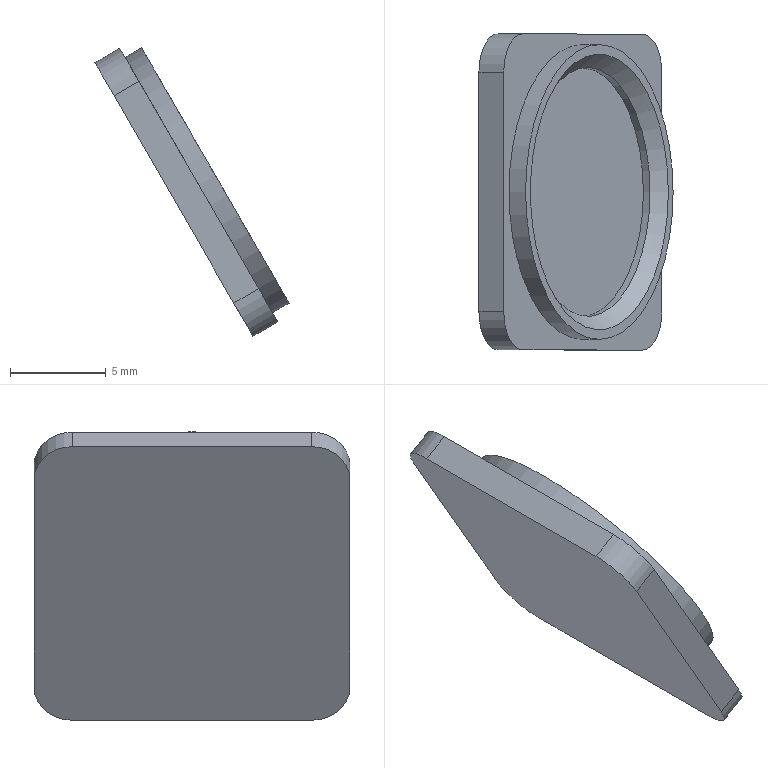Component | NX | ANALOG_FINGERPRINT_BUTTON | 1 solid | 15 faces | box 10.14 x 16.5 x 15.06 mm | volume 433 mm3 | plane 8 | cylinder 6 | cone 1 | commonest cylinder face diameters 4 x4 15.4 x1 13 x1
STEP:
#1=CARTESIAN_POINT('',(0.,0.,0.));
#2=DIRECTION('',(0.,0.,1.));
#3=DIRECTION('',(1.,0.,0.));
#4=AXIS2_PLACEMENT_3D('',#1,#2,#3);
#5=CARTESIAN_POINT('',(-17.256,7.851,157.651));
#6=VERTEX_POINT('',#5);
#7=CARTESIAN_POINT('',(-17.256,-4.649,157.651));
#8=VERTEX_POINT('',#7);
#9=CARTESIAN_POINT('',(-17.256,7.851,157.651));
#10=DIRECTION('',(0.,-1.,0.));
#11=VECTOR('',#10,1.);
#12=LINE('',#9,#11);
#13=CARTESIAN_POINT('',(-15.957,7.851,158.401));
#14=DIRECTION('',(0.5,0.,-0.866));
#15=DIRECTION('',(-0.866,0.,-0.5));
#16=AXIS2_PLACEMENT_3D('',#13,#14,#15);
#17=PLANE('',#16);
#18=CARTESIAN_POINT('',(1.5,0.));
#19=DIRECTION('',(0.,-1.));
#20=VECTOR('',#19,1.);
#21=LINE('',#18,#20);
#22=(GEOMETRIC_REPRESENTATION_CONTEXT(2)PARAMETRIC_REPRESENTATION_CONTEXT()REPRESENTATION_CONTEXT('',''));
#23=DEFINITIONAL_REPRESENTATION('',(#21),#22);
#24=PCURVE('',#17,#23);
#25=CARTESIAN_POINT('',(-16.256,-4.649,155.919));
#26=DIRECTION('',(0.866,0.,0.5));
#27=DIRECTION('',(0.5,0.,-0.866));
#28=AXIS2_PLACEMENT_3D('',#25,#26,#27);
#29=PLANE('',#28);
#30=CARTESIAN_POINT('',(-2.,12.5));
#31=DIRECTION('',(0.,-1.));
#32=VECTOR('',#31,1.);
#33=LINE('',#30,#32);
#34=(GEOMETRIC_REPRESENTATION_CONTEXT(2)PARAMETRIC_REPRESENTATION_CONTEXT()REPRESENTATION_CONTEXT('',''));
#35=DEFINITIONAL_REPRESENTATION('',(#33),#34);
#36=PCURVE('',#29,#35);
#37=SURFACE_CURVE('',#12,(#24,#36),.PCURVE_S1.);
#38=EDGE_CURVE('',#6,#8,#37,.T.);
#39=ORIENTED_EDGE('',*,*,#38,.T.);
#40=CARTESIAN_POINT('',(-15.957,-4.649,158.401));
#41=VERTEX_POINT('',#40);
#42=CARTESIAN_POINT('',(-15.957,-4.649,158.401));
#43=DIRECTION('',(-0.866,0.,-0.5));
#44=VECTOR('',#43,1.);
#45=LINE('',#42,#44);
#46=CARTESIAN_POINT('',(0.,-12.5));
#47=DIRECTION('',(1.,0.));
#48=VECTOR('',#47,1.);
#49=LINE('',#46,#48);
#50=(GEOMETRIC_REPRESENTATION_CONTEXT(2)PARAMETRIC_REPRESENTATION_CONTEXT()REPRESENTATION_CONTEXT('',''));
#51=DEFINITIONAL_REPRESENTATION('',(#49),#50);
#52=PCURVE('',#17,#51);
#53=CARTESIAN_POINT('',(-14.957,-4.649,156.669));
#54=DIRECTION('',(-0.866,0.,-0.5));
#55=DIRECTION('',(-0.5,0.,0.866));
#56=AXIS2_PLACEMENT_3D('',#53,#54,#55);
#57=CYLINDRICAL_SURFACE('',#56,2.);
#58=CARTESIAN_POINT('',(6.283,0.));
#59=DIRECTION('',(0.,1.));
#60=VECTOR('',#59,1.);
#61=LINE('',#58,#60);
#62=(GEOMETRIC_REPRESENTATION_CONTEXT(2)PARAMETRIC_REPRESENTATION_CONTEXT()REPRESENTATION_CONTEXT('',''));
#63=DEFINITIONAL_REPRESENTATION('',(#61),#62);
#64=PCURVE('',#57,#63);
#65=SURFACE_CURVE('',#45,(#52,#64),.PCURVE_S1.);
#66=EDGE_CURVE('',#41,#8,#65,.T.);
#67=ORIENTED_EDGE('',*,*,#66,.F.);
#68=CARTESIAN_POINT('',(-15.957,7.851,158.401));
#69=VERTEX_POINT('',#68);
#70=CARTESIAN_POINT('',(-15.957,7.851,158.401));
#71=DIRECTION('',(0.,-1.,0.));
#72=VECTOR('',#71,1.);
#73=LINE('',#70,#72);
#74=CARTESIAN_POINT('',(0.,0.));
#75=DIRECTION('',(0.,-1.));
#76=VECTOR('',#75,1.);
#77=LINE('',#74,#76);
#78=(GEOMETRIC_REPRESENTATION_CONTEXT(2)PARAMETRIC_REPRESENTATION_CONTEXT()REPRESENTATION_CONTEXT('',''));
#79=DEFINITIONAL_REPRESENTATION('',(#77),#78);
#80=PCURVE('',#17,#79);
#81=CARTESIAN_POINT('',(-14.957,-4.649,156.669));
#82=DIRECTION('',(0.866,0.,0.5));
#83=DIRECTION('',(0.5,0.,-0.866));
#84=AXIS2_PLACEMENT_3D('',#81,#82,#83);
#85=PLANE('',#84);
#86=CARTESIAN_POINT('',(-2.,12.5));
#87=DIRECTION('',(0.,-1.));
#88=VECTOR('',#87,1.);
#89=LINE('',#86,#88);
#90=(GEOMETRIC_REPRESENTATION_CONTEXT(2)PARAMETRIC_REPRESENTATION_CONTEXT()REPRESENTATION_CONTEXT('',''));
#91=DEFINITIONAL_REPRESENTATION('',(#89),#90);
#92=PCURVE('',#85,#91);
#93=SURFACE_CURVE('',#73,(#80,#92),.PCURVE_S1.);
#94=EDGE_CURVE('',#69,#41,#93,.T.);
#95=ORIENTED_EDGE('',*,*,#94,.F.);
#96=CARTESIAN_POINT('',(-15.957,7.851,158.401));
#97=DIRECTION('',(-0.866,0.,-0.5));
#98=VECTOR('',#97,1.);
#99=LINE('',#96,#98);
#100=CARTESIAN_POINT('',(0.,0.));
#101=DIRECTION('',(1.,0.));
#102=VECTOR('',#101,1.);
#103=LINE('',#100,#102);
#104=(GEOMETRIC_REPRESENTATION_CONTEXT(2)PARAMETRIC_REPRESENTATION_CONTEXT()REPRESENTATION_CONTEXT('',''));
#105=DEFINITIONAL_REPRESENTATION('',(#103),#104);
#106=PCURVE('',#17,#105);
#107=CARTESIAN_POINT('',(-14.957,7.851,156.669));
#108=DIRECTION('',(-0.866,0.,-0.5));
#109=DIRECTION('',(-0.5,0.,0.866));
#110=AXIS2_PLACEMENT_3D('',#107,#108,#109);
#111=CYLINDRICAL_SURFACE('',#110,2.);
#112=CARTESIAN_POINT('',(0.,0.));
#113=DIRECTION('',(0.,1.));
#114=VECTOR('',#113,1.);
#115=LINE('',#112,#114);
#116=(GEOMETRIC_REPRESENTATION_CONTEXT(2)PARAMETRIC_REPRESENTATION_CONTEXT()REPRESENTATION_CONTEXT('',''));
#117=DEFINITIONAL_REPRESENTATION('',(#115),#116);
#118=PCURVE('',#111,#117);
#119=SURFACE_CURVE('',#99,(#106,#118),.PCURVE_S1.);
#120=EDGE_CURVE('',#69,#6,#119,.T.);
#121=ORIENTED_EDGE('',*,*,#120,.T.);
#122=EDGE_LOOP('',(#39,#67,#95,#121));
#123=FACE_BOUND('',#122,.T.);
#124=ADVANCED_FACE('',(#123),#17,.F.);
#125=CARTESIAN_POINT('',(-16.256,-6.649,155.919));
#126=VERTEX_POINT('',#125);
#127=CARTESIAN_POINT('',(-16.256,-4.649,155.919));
#128=DIRECTION('',(0.866,0.,0.5));
#129=DIRECTION('',(0.5,0.,-0.866));
#130=AXIS2_PLACEMENT_3D('',#127,#128,#129);
#131=CIRCLE('',#130,2.);
#132=CARTESIAN_POINT('',(9.425,1.5));
#133=DIRECTION('',(-1.,-0.));
#134=VECTOR('',#133,1.);
#135=LINE('',#132,#134);
#136=(GEOMETRIC_REPRESENTATION_CONTEXT(2)PARAMETRIC_REPRESENTATION_CONTEXT()REPRESENTATION_CONTEXT('',''));
#137=DEFINITIONAL_REPRESENTATION('',(#135),#136);
#138=PCURVE('',#57,#137);
#139=CARTESIAN_POINT('',(0.,0.));
#140=DIRECTION('',(1.,0.));
#141=AXIS2_PLACEMENT_2D('',#139,#140);
#142=CIRCLE('',#141,2.);
#143=(GEOMETRIC_REPRESENTATION_CONTEXT(2)PARAMETRIC_REPRESENTATION_CONTEXT()REPRESENTATION_CONTEXT('',''));
#144=DEFINITIONAL_REPRESENTATION('',(#142),#143);
#145=PCURVE('',#29,#144);
#146=SURFACE_CURVE('',#131,(#138,#145),.PCURVE_S1.);
#147=EDGE_CURVE('',#8,#126,#146,.T.);
#148=ORIENTED_EDGE('',*,*,#147,.T.);
#149=CARTESIAN_POINT('',(-14.957,-6.649,156.669));
#150=VERTEX_POINT('',#149);
#151=CARTESIAN_POINT('',(-14.957,-6.649,156.669));
#152=DIRECTION('',(-0.866,0.,-0.5));
#153=VECTOR('',#152,1.);
#154=LINE('',#151,#153);
#155=CARTESIAN_POINT('',(4.712,0.));
#156=DIRECTION('',(0.,1.));
#157=VECTOR('',#156,1.);
#158=LINE('',#155,#157);
#159=(GEOMETRIC_REPRESENTATION_CONTEXT(2)PARAMETRIC_REPRESENTATION_CONTEXT()REPRESENTATION_CONTEXT('',''));
#160=DEFINITIONAL_REPRESENTATION('',(#158),#159);
#161=PCURVE('',#57,#160);
#162=CARTESIAN_POINT('',(-14.957,-6.649,156.669));
#163=DIRECTION('',(0.,1.,0.));
#164=DIRECTION('',(0.866,0.,0.5));
#165=AXIS2_PLACEMENT_3D('',#162,#163,#164);
#166=PLANE('',#165);
#167=CARTESIAN_POINT('',(0.,0.));
#168=DIRECTION('',(-1.,0.));
#169=VECTOR('',#168,1.);
#170=LINE('',#167,#169);
#171=(GEOMETRIC_REPRESENTATION_CONTEXT(2)PARAMETRIC_REPRESENTATION_CONTEXT()REPRESENTATION_CONTEXT('',''));
#172=DEFINITIONAL_REPRESENTATION('',(#170),#171);
#173=PCURVE('',#166,#172);
#174=SURFACE_CURVE('',#154,(#161,#173),.PCURVE_S1.);
#175=EDGE_CURVE('',#150,#126,#174,.T.);
#176=ORIENTED_EDGE('',*,*,#175,.F.);
#177=CARTESIAN_POINT('',(-14.957,-4.649,156.669));
#178=DIRECTION('',(0.866,0.,0.5));
#179=DIRECTION('',(0.5,0.,-0.866));
#180=AXIS2_PLACEMENT_3D('',#177,#178,#179);
#181=CIRCLE('',#180,2.);
#182=CARTESIAN_POINT('',(9.425,0.));
#183=DIRECTION('',(-1.,0.));
#184=VECTOR('',#183,1.);
#185=LINE('',#182,#184);
#186=(GEOMETRIC_REPRESENTATION_CONTEXT(2)PARAMETRIC_REPRESENTATION_CONTEXT()REPRESENTATION_CONTEXT('',''));
#187=DEFINITIONAL_REPRESENTATION('',(#185),#186);
#188=PCURVE('',#57,#187);
#189=CARTESIAN_POINT('',(0.,0.));
#190=DIRECTION('',(1.,0.));
#191=AXIS2_PLACEMENT_2D('',#189,#190);
#192=CIRCLE('',#191,2.);
#193=(GEOMETRIC_REPRESENTATION_CONTEXT(2)PARAMETRIC_REPRESENTATION_CONTEXT()REPRESENTATION_CONTEXT('',''));
#194=DEFINITIONAL_REPRESENTATION('',(#192),#193);
#195=PCURVE('',#85,#194);
#196=SURFACE_CURVE('',#181,(#188,#195),.PCURVE_S1.);
#197=EDGE_CURVE('',#41,#150,#196,.T.);
#198=ORIENTED_EDGE('',*,*,#197,.F.);
#199=ORIENTED_EDGE('',*,*,#66,.T.);
#200=EDGE_LOOP('',(#148,#176,#198,#199));
#201=FACE_BOUND('',#200,.T.);
#202=ADVANCED_FACE('',(#201),#57,.T.);
#203=CARTESIAN_POINT('',(-10.006,-6.649,145.094));
#204=VERTEX_POINT('',#203);
#205=CARTESIAN_POINT('',(-16.256,-6.649,155.919));
#206=DIRECTION('',(0.5,0.,-0.866));
#207=VECTOR('',#206,1.);
#208=LINE('',#205,#207);
#209=CARTESIAN_POINT('',(-1.5,0.));
#210=DIRECTION('',(0.,1.));
#211=VECTOR('',#210,1.);
#212=LINE('',#209,#211);
#213=(GEOMETRIC_REPRESENTATION_CONTEXT(2)PARAMETRIC_REPRESENTATION_CONTEXT()REPRESENTATION_CONTEXT('',''));
#214=DEFINITIONAL_REPRESENTATION('',(#212),#213);
#215=PCURVE('',#166,#214);
#216=CARTESIAN_POINT('',(0.,-2.));
#217=DIRECTION('',(1.,0.));
#218=VECTOR('',#217,1.);
#219=LINE('',#216,#218);
#220=(GEOMETRIC_REPRESENTATION_CONTEXT(2)PARAMETRIC_REPRESENTATION_CONTEXT()REPRESENTATION_CONTEXT('',''));
#221=DEFINITIONAL_REPRESENTATION('',(#219),#220);
#222=PCURVE('',#29,#221);
#223=SURFACE_CURVE('',#208,(#215,#222),.PCURVE_S1.);
#224=EDGE_CURVE('',#126,#204,#223,.T.);
#225=ORIENTED_EDGE('',*,*,#224,.T.);
#226=CARTESIAN_POINT('',(-8.707,-6.649,145.844));
#227=VERTEX_POINT('',#226);
#228=CARTESIAN_POINT('',(-8.707,-6.649,145.844));
#229=DIRECTION('',(-0.866,0.,-0.5));
#230=VECTOR('',#229,1.);
#231=LINE('',#228,#230);
#232=CARTESIAN_POINT('',(-0.,12.5));
#233=DIRECTION('',(-1.,0.));
#234=VECTOR('',#233,1.);
#235=LINE('',#232,#234);
#236=(GEOMETRIC_REPRESENTATION_CONTEXT(2)PARAMETRIC_REPRESENTATION_CONTEXT()REPRESENTATION_CONTEXT('',''));
#237=DEFINITIONAL_REPRESENTATION('',(#235),#236);
#238=PCURVE('',#166,#237);
#239=CARTESIAN_POINT('',(-8.707,-4.649,145.844));
#240=DIRECTION('',(-0.866,0.,-0.5));
#241=DIRECTION('',(-0.5,0.,0.866));
#242=AXIS2_PLACEMENT_3D('',#239,#240,#241);
#243=CYLINDRICAL_SURFACE('',#242,2.);
#244=CARTESIAN_POINT('',(4.712,0.));
#245=DIRECTION('',(0.,1.));
#246=VECTOR('',#245,1.);
#247=LINE('',#244,#246);
#248=(GEOMETRIC_REPRESENTATION_CONTEXT(2)PARAMETRIC_REPRESENTATION_CONTEXT()REPRESENTATION_CONTEXT('',''));
#249=DEFINITIONAL_REPRESENTATION('',(#247),#248);
#250=PCURVE('',#243,#249);
#251=SURFACE_CURVE('',#231,(#238,#250),.PCURVE_S1.);
#252=EDGE_CURVE('',#227,#204,#251,.T.);
#253=ORIENTED_EDGE('',*,*,#252,.F.);
#254=CARTESIAN_POINT('',(-14.957,-6.649,156.669));
#255=DIRECTION('',(0.5,0.,-0.866));
#256=VECTOR('',#255,1.);
#257=LINE('',#254,#256);
#258=CARTESIAN_POINT('',(0.,0.));
#259=DIRECTION('',(0.,1.));
#260=VECTOR('',#259,1.);
#261=LINE('',#258,#260);
#262=(GEOMETRIC_REPRESENTATION_CONTEXT(2)PARAMETRIC_REPRESENTATION_CONTEXT()REPRESENTATION_CONTEXT('',''));
#263=DEFINITIONAL_REPRESENTATION('',(#261),#262);
#264=PCURVE('',#166,#263);
#265=CARTESIAN_POINT('',(0.,-2.));
#266=DIRECTION('',(1.,0.));
#267=VECTOR('',#266,1.);
#268=LINE('',#265,#267);
#269=(GEOMETRIC_REPRESENTATION_CONTEXT(2)PARAMETRIC_REPRESENTATION_CONTEXT()REPRESENTATION_CONTEXT('',''));
#270=DEFINITIONAL_REPRESENTATION('',(#268),#269);
#271=PCURVE('',#85,#270);
#272=SURFACE_CURVE('',#257,(#264,#271),.PCURVE_S1.);
#273=EDGE_CURVE('',#150,#227,#272,.T.);
#274=ORIENTED_EDGE('',*,*,#273,.F.);
#275=ORIENTED_EDGE('',*,*,#175,.T.);
#276=EDGE_LOOP('',(#225,#253,#274,#275));
#277=FACE_BOUND('',#276,.T.);
#278=ADVANCED_FACE('',(#277),#166,.F.);
#279=CARTESIAN_POINT('',(-9.006,-4.649,143.362));
#280=VERTEX_POINT('',#279);
#281=CARTESIAN_POINT('',(-10.006,-4.649,145.094));
#282=DIRECTION('',(0.866,0.,0.5));
#283=DIRECTION('',(0.5,0.,-0.866));
#284=AXIS2_PLACEMENT_3D('',#281,#282,#283);
#285=CIRCLE('',#284,2.);
#286=CARTESIAN_POINT('',(9.425,1.5));
#287=DIRECTION('',(-1.,0.));
#288=VECTOR('',#287,1.);
#289=LINE('',#286,#288);
#290=(GEOMETRIC_REPRESENTATION_CONTEXT(2)PARAMETRIC_REPRESENTATION_CONTEXT()REPRESENTATION_CONTEXT('',''));
#291=DEFINITIONAL_REPRESENTATION('',(#289),#290);
#292=PCURVE('',#243,#291);
#293=CARTESIAN_POINT('',(12.5,0.));
#294=DIRECTION('',(1.,0.));
#295=AXIS2_PLACEMENT_2D('',#293,#294);
#296=CIRCLE('',#295,2.);
#297=(GEOMETRIC_REPRESENTATION_CONTEXT(2)PARAMETRIC_REPRESENTATION_CONTEXT()REPRESENTATION_CONTEXT('',''));
#298=DEFINITIONAL_REPRESENTATION('',(#296),#297);
#299=PCURVE('',#29,#298);
#300=SURFACE_CURVE('',#285,(#292,#299),.PCURVE_S1.);
#301=EDGE_CURVE('',#204,#280,#300,.T.);
#302=ORIENTED_EDGE('',*,*,#301,.T.);
#303=CARTESIAN_POINT('',(-7.707,-4.649,144.112));
#304=VERTEX_POINT('',#303);
#305=CARTESIAN_POINT('',(-7.707,-4.649,144.112));
#306=DIRECTION('',(-0.866,0.,-0.5));
#307=VECTOR('',#306,1.);
#308=LINE('',#305,#307);
#309=CARTESIAN_POINT('',(3.142,0.));
#310=DIRECTION('',(0.,1.));
#311=VECTOR('',#310,1.);
#312=LINE('',#309,#311);
#313=(GEOMETRIC_REPRESENTATION_CONTEXT(2)PARAMETRIC_REPRESENTATION_CONTEXT()REPRESENTATION_CONTEXT('',''));
#314=DEFINITIONAL_REPRESENTATION('',(#312),#313);
#315=PCURVE('',#243,#314);
#316=CARTESIAN_POINT('',(-7.707,-4.649,144.112));
#317=DIRECTION('',(-0.5,0.,0.866));
#318=DIRECTION('',(0.866,0.,0.5));
#319=AXIS2_PLACEMENT_3D('',#316,#317,#318);
#320=PLANE('',#319);
#321=CARTESIAN_POINT('',(0.,0.));
#322=DIRECTION('',(-1.,0.));
#323=VECTOR('',#322,1.);
#324=LINE('',#321,#323);
#325=(GEOMETRIC_REPRESENTATION_CONTEXT(2)PARAMETRIC_REPRESENTATION_CONTEXT()REPRESENTATION_CONTEXT('',''));
#326=DEFINITIONAL_REPRESENTATION('',(#324),#325);
#327=PCURVE('',#320,#326);
#328=SURFACE_CURVE('',#308,(#315,#327),.PCURVE_S1.);
#329=EDGE_CURVE('',#304,#280,#328,.T.);
#330=ORIENTED_EDGE('',*,*,#329,.F.);
#331=CARTESIAN_POINT('',(-8.707,-4.649,145.844));
#332=DIRECTION('',(0.866,0.,0.5));
#333=DIRECTION('',(0.5,0.,-0.866));
#334=AXIS2_PLACEMENT_3D('',#331,#332,#333);
#335=CIRCLE('',#334,2.);
#336=CARTESIAN_POINT('',(9.425,0.));
#337=DIRECTION('',(-1.,-0.));
#338=VECTOR('',#337,1.);
#339=LINE('',#336,#338);
#340=(GEOMETRIC_REPRESENTATION_CONTEXT(2)PARAMETRIC_REPRESENTATION_CONTEXT()REPRESENTATION_CONTEXT('',''));
#341=DEFINITIONAL_REPRESENTATION('',(#339),#340);
#342=PCURVE('',#243,#341);
#343=CARTESIAN_POINT('',(12.5,0.));
#344=DIRECTION('',(1.,0.));
#345=AXIS2_PLACEMENT_2D('',#343,#344);
#346=CIRCLE('',#345,2.);
#347=(GEOMETRIC_REPRESENTATION_CONTEXT(2)PARAMETRIC_REPRESENTATION_CONTEXT()REPRESENTATION_CONTEXT('',''));
#348=DEFINITIONAL_REPRESENTATION('',(#346),#347);
#349=PCURVE('',#85,#348);
#350=SURFACE_CURVE('',#335,(#342,#349),.PCURVE_S1.);
#351=EDGE_CURVE('',#227,#304,#350,.T.);
#352=ORIENTED_EDGE('',*,*,#351,.F.);
#353=ORIENTED_EDGE('',*,*,#252,.T.);
#354=EDGE_LOOP('',(#302,#330,#352,#353));
#355=FACE_BOUND('',#354,.T.);
#356=ADVANCED_FACE('',(#355),#243,.T.);
#357=CARTESIAN_POINT('',(-9.006,7.851,143.362));
#358=VERTEX_POINT('',#357);
#359=CARTESIAN_POINT('',(-9.006,-4.649,143.362));
#360=DIRECTION('',(0.,1.,0.));
#361=VECTOR('',#360,1.);
#362=LINE('',#359,#361);
#363=CARTESIAN_POINT('',(-1.5,0.));
#364=DIRECTION('',(0.,1.));
#365=VECTOR('',#364,1.);
#366=LINE('',#363,#365);
#367=(GEOMETRIC_REPRESENTATION_CONTEXT(2)PARAMETRIC_REPRESENTATION_CONTEXT()REPRESENTATION_CONTEXT('',''));
#368=DEFINITIONAL_REPRESENTATION('',(#366),#367);
#369=PCURVE('',#320,#368);
#370=CARTESIAN_POINT('',(14.5,0.));
#371=DIRECTION('',(0.,1.));
#372=VECTOR('',#371,1.);
#373=LINE('',#370,#372);
#374=(GEOMETRIC_REPRESENTATION_CONTEXT(2)PARAMETRIC_REPRESENTATION_CONTEXT()REPRESENTATION_CONTEXT('',''));
#375=DEFINITIONAL_REPRESENTATION('',(#373),#374);
#376=PCURVE('',#29,#375);
#377=SURFACE_CURVE('',#362,(#369,#376),.PCURVE_S1.);
#378=EDGE_CURVE('',#280,#358,#377,.T.);
#379=ORIENTED_EDGE('',*,*,#378,.T.);
#380=CARTESIAN_POINT('',(-7.707,7.851,144.112));
#381=VERTEX_POINT('',#380);
#382=CARTESIAN_POINT('',(-7.707,7.851,144.112));
#383=DIRECTION('',(-0.866,0.,-0.5));
#384=VECTOR('',#383,1.);
#385=LINE('',#382,#384);
#386=CARTESIAN_POINT('',(0.,12.5));
#387=DIRECTION('',(-1.,0.));
#388=VECTOR('',#387,1.);
#389=LINE('',#386,#388);
#390=(GEOMETRIC_REPRESENTATION_CONTEXT(2)PARAMETRIC_REPRESENTATION_CONTEXT()REPRESENTATION_CONTEXT('',''));
#391=DEFINITIONAL_REPRESENTATION('',(#389),#390);
#392=PCURVE('',#320,#391);
#393=CARTESIAN_POINT('',(-8.707,7.851,145.844));
#394=DIRECTION('',(-0.866,0.,-0.5));
#395=DIRECTION('',(-0.5,0.,0.866));
#396=AXIS2_PLACEMENT_3D('',#393,#394,#395);
#397=CYLINDRICAL_SURFACE('',#396,2.);
#398=CARTESIAN_POINT('',(3.142,0.));
#399=DIRECTION('',(0.,1.));
#400=VECTOR('',#399,1.);
#401=LINE('',#398,#400);
#402=(GEOMETRIC_REPRESENTATION_CONTEXT(2)PARAMETRIC_REPRESENTATION_CONTEXT()REPRESENTATION_CONTEXT('',''));
#403=DEFINITIONAL_REPRESENTATION('',(#401),#402);
#404=PCURVE('',#397,#403);
#405=SURFACE_CURVE('',#385,(#392,#404),.PCURVE_S1.);
#406=EDGE_CURVE('',#381,#358,#405,.T.);
#407=ORIENTED_EDGE('',*,*,#406,.F.);
#408=CARTESIAN_POINT('',(-7.707,-4.649,144.112));
#409=DIRECTION('',(0.,1.,0.));
#410=VECTOR('',#409,1.);
#411=LINE('',#408,#410);
#412=CARTESIAN_POINT('',(0.,0.));
#413=DIRECTION('',(0.,1.));
#414=VECTOR('',#413,1.);
#415=LINE('',#412,#414);
#416=(GEOMETRIC_REPRESENTATION_CONTEXT(2)PARAMETRIC_REPRESENTATION_CONTEXT()REPRESENTATION_CONTEXT('',''));
#417=DEFINITIONAL_REPRESENTATION('',(#415),#416);
#418=PCURVE('',#320,#417);
#419=CARTESIAN_POINT('',(14.5,0.));
#420=DIRECTION('',(0.,1.));
#421=VECTOR('',#420,1.);
#422=LINE('',#419,#421);
#423=(GEOMETRIC_REPRESENTATION_CONTEXT(2)PARAMETRIC_REPRESENTATION_CONTEXT()REPRESENTATION_CONTEXT('',''));
#424=DEFINITIONAL_REPRESENTATION('',(#422),#423);
#425=PCURVE('',#85,#424);
#426=SURFACE_CURVE('',#411,(#418,#425),.PCURVE_S1.);
#427=EDGE_CURVE('',#304,#381,#426,.T.);
#428=ORIENTED_EDGE('',*,*,#427,.F.);
#429=ORIENTED_EDGE('',*,*,#329,.T.);
#430=EDGE_LOOP('',(#379,#407,#428,#429));
#431=FACE_BOUND('',#430,.T.);
#432=ADVANCED_FACE('',(#431),#320,.F.);
#433=CARTESIAN_POINT('',(-10.006,9.851,145.094));
#434=VERTEX_POINT('',#433);
#435=CARTESIAN_POINT('',(-10.006,7.851,145.094));
#436=DIRECTION('',(0.866,0.,0.5));
#437=DIRECTION('',(0.5,0.,-0.866));
#438=AXIS2_PLACEMENT_3D('',#435,#436,#437);
#439=CIRCLE('',#438,2.);
#440=CARTESIAN_POINT('',(3.142,1.5));
#441=DIRECTION('',(-1.,0.));
#442=VECTOR('',#441,1.);
#443=LINE('',#440,#442);
#444=(GEOMETRIC_REPRESENTATION_CONTEXT(2)PARAMETRIC_REPRESENTATION_CONTEXT()REPRESENTATION_CONTEXT('',''));
#445=DEFINITIONAL_REPRESENTATION('',(#443),#444);
#446=PCURVE('',#397,#445);
#447=CARTESIAN_POINT('',(12.5,12.5));
#448=DIRECTION('',(1.,0.));
#449=AXIS2_PLACEMENT_2D('',#447,#448);
#450=CIRCLE('',#449,2.);
#451=(GEOMETRIC_REPRESENTATION_CONTEXT(2)PARAMETRIC_REPRESENTATION_CONTEXT()REPRESENTATION_CONTEXT('',''));
#452=DEFINITIONAL_REPRESENTATION('',(#450),#451);
#453=PCURVE('',#29,#452);
#454=SURFACE_CURVE('',#439,(#446,#453),.PCURVE_S1.);
#455=EDGE_CURVE('',#358,#434,#454,.T.);
#456=ORIENTED_EDGE('',*,*,#455,.T.);
#457=CARTESIAN_POINT('',(-8.707,9.851,145.844));
#458=VERTEX_POINT('',#457);
#459=CARTESIAN_POINT('',(-8.707,9.851,145.844));
#460=DIRECTION('',(-0.866,0.,-0.5));
#461=VECTOR('',#460,1.);
#462=LINE('',#459,#461);
#463=CARTESIAN_POINT('',(1.571,0.));
#464=DIRECTION('',(-0.,1.));
#465=VECTOR('',#464,1.);
#466=LINE('',#463,#465);
#467=(GEOMETRIC_REPRESENTATION_CONTEXT(2)PARAMETRIC_REPRESENTATION_CONTEXT()REPRESENTATION_CONTEXT('',''));
#468=DEFINITIONAL_REPRESENTATION('',(#466),#467);
#469=PCURVE('',#397,#468);
#470=CARTESIAN_POINT('',(-8.707,9.851,145.844));
#471=DIRECTION('',(0.,-1.,0.));
#472=DIRECTION('',(-0.866,0.,-0.5));
#473=AXIS2_PLACEMENT_3D('',#470,#471,#472);
#474=PLANE('',#473);
#475=CARTESIAN_POINT('',(0.,0.));
#476=DIRECTION('',(1.,0.));
#477=VECTOR('',#476,1.);
#478=LINE('',#475,#477);
#479=(GEOMETRIC_REPRESENTATION_CONTEXT(2)PARAMETRIC_REPRESENTATION_CONTEXT()REPRESENTATION_CONTEXT('',''));
#480=DEFINITIONAL_REPRESENTATION('',(#478),#479);
#481=PCURVE('',#474,#480);
#482=SURFACE_CURVE('',#462,(#469,#481),.PCURVE_S1.);
#483=EDGE_CURVE('',#458,#434,#482,.T.);
#484=ORIENTED_EDGE('',*,*,#483,.F.);
#485=CARTESIAN_POINT('',(-8.707,7.851,145.844));
#486=DIRECTION('',(0.866,0.,0.5));
#487=DIRECTION('',(0.5,0.,-0.866));
#488=AXIS2_PLACEMENT_3D('',#485,#486,#487);
#489=CIRCLE('',#488,2.);
#490=CARTESIAN_POINT('',(3.142,-0.));
#491=DIRECTION('',(-1.,0.));
#492=VECTOR('',#491,1.);
#493=LINE('',#490,#492);
#494=(GEOMETRIC_REPRESENTATION_CONTEXT(2)PARAMETRIC_REPRESENTATION_CONTEXT()REPRESENTATION_CONTEXT('',''));
#495=DEFINITIONAL_REPRESENTATION('',(#493),#494);
#496=PCURVE('',#397,#495);
#497=CARTESIAN_POINT('',(12.5,12.5));
#498=DIRECTION('',(1.,0.));
#499=AXIS2_PLACEMENT_2D('',#497,#498);
#500=CIRCLE('',#499,2.);
#501=(GEOMETRIC_REPRESENTATION_CONTEXT(2)PARAMETRIC_REPRESENTATION_CONTEXT()REPRESENTATION_CONTEXT('',''));
#502=DEFINITIONAL_REPRESENTATION('',(#500),#501);
#503=PCURVE('',#85,#502);
#504=SURFACE_CURVE('',#489,(#496,#503),.PCURVE_S1.);
#505=EDGE_CURVE('',#381,#458,#504,.T.);
#506=ORIENTED_EDGE('',*,*,#505,.F.);
#507=ORIENTED_EDGE('',*,*,#406,.T.);
#508=EDGE_LOOP('',(#456,#484,#506,#507));
#509=FACE_BOUND('',#508,.T.);
#510=ADVANCED_FACE('',(#509),#397,.T.);
#511=CARTESIAN_POINT('',(-16.256,9.851,155.919));
#512=VERTEX_POINT('',#511);
#513=CARTESIAN_POINT('',(-10.006,9.851,145.094));
#514=DIRECTION('',(-0.5,0.,0.866));
#515=VECTOR('',#514,1.);
#516=LINE('',#513,#515);
#517=CARTESIAN_POINT('',(1.5,0.));
#518=DIRECTION('',(0.,-1.));
#519=VECTOR('',#518,1.);
#520=LINE('',#517,#519);
#521=(GEOMETRIC_REPRESENTATION_CONTEXT(2)PARAMETRIC_REPRESENTATION_CONTEXT()REPRESENTATION_CONTEXT('',''));
#522=DEFINITIONAL_REPRESENTATION('',(#520),#521);
#523=PCURVE('',#474,#522);
#524=CARTESIAN_POINT('',(12.5,14.5));
#525=DIRECTION('',(-1.,0.));
#526=VECTOR('',#525,1.);
#527=LINE('',#524,#526);
#528=(GEOMETRIC_REPRESENTATION_CONTEXT(2)PARAMETRIC_REPRESENTATION_CONTEXT()REPRESENTATION_CONTEXT('',''));
#529=DEFINITIONAL_REPRESENTATION('',(#527),#528);
#530=PCURVE('',#29,#529);
#531=SURFACE_CURVE('',#516,(#523,#530),.PCURVE_S1.);
#532=EDGE_CURVE('',#434,#512,#531,.T.);
#533=ORIENTED_EDGE('',*,*,#532,.T.);
#534=CARTESIAN_POINT('',(-14.957,9.851,156.669));
#535=VERTEX_POINT('',#534);
#536=CARTESIAN_POINT('',(-14.957,9.851,156.669));
#537=DIRECTION('',(-0.866,0.,-0.5));
#538=VECTOR('',#537,1.);
#539=LINE('',#536,#538);
#540=CARTESIAN_POINT('',(-0.,-12.5));
#541=DIRECTION('',(1.,0.));
#542=VECTOR('',#541,1.);
#543=LINE('',#540,#542);
#544=(GEOMETRIC_REPRESENTATION_CONTEXT(2)PARAMETRIC_REPRESENTATION_CONTEXT()REPRESENTATION_CONTEXT('',''));
#545=DEFINITIONAL_REPRESENTATION('',(#543),#544);
#546=PCURVE('',#474,#545);
#547=CARTESIAN_POINT('',(1.571,0.));
#548=DIRECTION('',(0.,1.));
#549=VECTOR('',#548,1.);
#550=LINE('',#547,#549);
#551=(GEOMETRIC_REPRESENTATION_CONTEXT(2)PARAMETRIC_REPRESENTATION_CONTEXT()REPRESENTATION_CONTEXT('',''));
#552=DEFINITIONAL_REPRESENTATION('',(#550),#551);
#553=PCURVE('',#111,#552);
#554=SURFACE_CURVE('',#539,(#546,#553),.PCURVE_S1.);
#555=EDGE_CURVE('',#535,#512,#554,.T.);
#556=ORIENTED_EDGE('',*,*,#555,.F.);
#557=CARTESIAN_POINT('',(-8.707,9.851,145.844));
#558=DIRECTION('',(-0.5,0.,0.866));
#559=VECTOR('',#558,1.);
#560=LINE('',#557,#559);
#561=CARTESIAN_POINT('',(0.,0.));
#562=DIRECTION('',(0.,-1.));
#563=VECTOR('',#562,1.);
#564=LINE('',#561,#563);
#565=(GEOMETRIC_REPRESENTATION_CONTEXT(2)PARAMETRIC_REPRESENTATION_CONTEXT()REPRESENTATION_CONTEXT('',''));
#566=DEFINITIONAL_REPRESENTATION('',(#564),#565);
#567=PCURVE('',#474,#566);
#568=CARTESIAN_POINT('',(12.5,14.5));
#569=DIRECTION('',(-1.,0.));
#570=VECTOR('',#569,1.);
#571=LINE('',#568,#570);
#572=(GEOMETRIC_REPRESENTATION_CONTEXT(2)PARAMETRIC_REPRESENTATION_CONTEXT()REPRESENTATION_CONTEXT('',''));
#573=DEFINITIONAL_REPRESENTATION('',(#571),#572);
#574=PCURVE('',#85,#573);
#575=SURFACE_CURVE('',#560,(#567,#574),.PCURVE_S1.);
#576=EDGE_CURVE('',#458,#535,#575,.T.);
#577=ORIENTED_EDGE('',*,*,#576,.F.);
#578=ORIENTED_EDGE('',*,*,#483,.T.);
#579=EDGE_LOOP('',(#533,#556,#577,#578));
#580=FACE_BOUND('',#579,.T.);
#581=ADVANCED_FACE('',(#580),#474,.F.);
#582=CARTESIAN_POINT('',(-16.256,7.851,155.919));
#583=DIRECTION('',(0.866,0.,0.5));
#584=DIRECTION('',(0.5,0.,-0.866));
#585=AXIS2_PLACEMENT_3D('',#582,#583,#584);
#586=CIRCLE('',#585,2.);
#587=CARTESIAN_POINT('',(3.142,1.5));
#588=DIRECTION('',(-1.,0.));
#589=VECTOR('',#588,1.);
#590=LINE('',#587,#589);
#591=(GEOMETRIC_REPRESENTATION_CONTEXT(2)PARAMETRIC_REPRESENTATION_CONTEXT()REPRESENTATION_CONTEXT('',''));
#592=DEFINITIONAL_REPRESENTATION('',(#590),#591);
#593=PCURVE('',#111,#592);
#594=CARTESIAN_POINT('',(0.,12.5));
#595=DIRECTION('',(1.,0.));
#596=AXIS2_PLACEMENT_2D('',#594,#595);
#597=CIRCLE('',#596,2.);
#598=(GEOMETRIC_REPRESENTATION_CONTEXT(2)PARAMETRIC_REPRESENTATION_CONTEXT()REPRESENTATION_CONTEXT('',''));
#599=DEFINITIONAL_REPRESENTATION('',(#597),#598);
#600=PCURVE('',#29,#599);
#601=SURFACE_CURVE('',#586,(#593,#600),.PCURVE_S1.);
#602=EDGE_CURVE('',#512,#6,#601,.T.);
#603=ORIENTED_EDGE('',*,*,#602,.T.);
#604=ORIENTED_EDGE('',*,*,#120,.F.);
#605=CARTESIAN_POINT('',(-14.957,7.851,156.669));
#606=DIRECTION('',(0.866,0.,0.5));
#607=DIRECTION('',(0.5,0.,-0.866));
#608=AXIS2_PLACEMENT_3D('',#605,#606,#607);
#609=CIRCLE('',#608,2.);
#610=CARTESIAN_POINT('',(3.142,0.));
#611=DIRECTION('',(-1.,0.));
#612=VECTOR('',#611,1.);
#613=LINE('',#610,#612);
#614=(GEOMETRIC_REPRESENTATION_CONTEXT(2)PARAMETRIC_REPRESENTATION_CONTEXT()REPRESENTATION_CONTEXT('',''));
#615=DEFINITIONAL_REPRESENTATION('',(#613),#614);
#616=PCURVE('',#111,#615);
#617=CARTESIAN_POINT('',(0.,12.5));
#618=DIRECTION('',(1.,0.));
#619=AXIS2_PLACEMENT_2D('',#617,#618);
#620=CIRCLE('',#619,2.);
#621=(GEOMETRIC_REPRESENTATION_CONTEXT(2)PARAMETRIC_REPRESENTATION_CONTEXT()REPRESENTATION_CONTEXT('',''));
#622=DEFINITIONAL_REPRESENTATION('',(#620),#621);
#623=PCURVE('',#85,#622);
#624=SURFACE_CURVE('',#609,(#616,#623),.PCURVE_S1.);
#625=EDGE_CURVE('',#535,#69,#624,.T.);
#626=ORIENTED_EDGE('',*,*,#625,.F.);
#627=ORIENTED_EDGE('',*,*,#555,.T.);
#628=EDGE_LOOP('',(#603,#604,#626,#627));
#629=FACE_BOUND('',#628,.T.);
#630=ADVANCED_FACE('',(#629),#111,.T.);
#631=CARTESIAN_POINT('',(-7.982,1.601,144.588));
#632=VERTEX_POINT('',#631);
#633=CARTESIAN_POINT('',(-11.832,1.601,151.257));
#634=DIRECTION('',(0.866,0.,0.5));
#635=DIRECTION('',(0.5,0.,-0.866));
#636=AXIS2_PLACEMENT_3D('',#633,#634,#635);
#637=CIRCLE('',#636,7.7);
#638=CARTESIAN_POINT('',(6.25,6.25));
#639=DIRECTION('',(1.,0.));
#640=AXIS2_PLACEMENT_2D('',#638,#639);
#641=CIRCLE('',#640,7.7);
#642=(GEOMETRIC_REPRESENTATION_CONTEXT(2)PARAMETRIC_REPRESENTATION_CONTEXT()REPRESENTATION_CONTEXT('',''));
#643=DEFINITIONAL_REPRESENTATION('',(#641),#642);
#644=PCURVE('',#85,#643);
#645=CARTESIAN_POINT('',(-13.131,1.601,150.507));
#646=DIRECTION('',(0.866,0.,0.5));
#647=DIRECTION('',(0.5,0.,-0.866));
#648=AXIS2_PLACEMENT_3D('',#645,#646,#647);
#649=CYLINDRICAL_SURFACE('',#648,7.7);
#650=CARTESIAN_POINT('',(0.,1.5));
#651=DIRECTION('',(1.,0.));
#652=VECTOR('',#651,1.);
#653=LINE('',#650,#652);
#654=(GEOMETRIC_REPRESENTATION_CONTEXT(2)PARAMETRIC_REPRESENTATION_CONTEXT()REPRESENTATION_CONTEXT('',''));
#655=DEFINITIONAL_REPRESENTATION('',(#653),#654);
#656=PCURVE('',#649,#655);
#657=SURFACE_CURVE('',#637,(#644,#656),.PCURVE_S1.);
#658=EDGE_CURVE('',#632,#632,#657,.T.);
#659=ORIENTED_EDGE('',*,*,#658,.F.);
#660=EDGE_LOOP('',(#659));
#661=FACE_BOUND('',#660,.T.);
#662=ORIENTED_EDGE('',*,*,#94,.T.);
#663=ORIENTED_EDGE('',*,*,#197,.T.);
#664=ORIENTED_EDGE('',*,*,#273,.T.);
#665=ORIENTED_EDGE('',*,*,#351,.T.);
#666=ORIENTED_EDGE('',*,*,#427,.T.);
#667=ORIENTED_EDGE('',*,*,#505,.T.);
#668=ORIENTED_EDGE('',*,*,#576,.T.);
#669=ORIENTED_EDGE('',*,*,#625,.T.);
#670=EDGE_LOOP('',(#662,#663,#664,#665,#666,#667,#668,#669));
#671=FACE_BOUND('',#670,.T.);
#672=ADVANCED_FACE('',(#661,#671),#85,.T.);
#673=ORIENTED_EDGE('',*,*,#38,.F.);
#674=ORIENTED_EDGE('',*,*,#602,.F.);
#675=ORIENTED_EDGE('',*,*,#532,.F.);
#676=ORIENTED_EDGE('',*,*,#455,.F.);
#677=ORIENTED_EDGE('',*,*,#378,.F.);
#678=ORIENTED_EDGE('',*,*,#301,.F.);
#679=ORIENTED_EDGE('',*,*,#224,.F.);
#680=ORIENTED_EDGE('',*,*,#147,.F.);
#681=EDGE_LOOP('',(#673,#674,#675,#676,#677,#678,#679,#680));
#682=FACE_BOUND('',#681,.T.);
#683=ADVANCED_FACE('',(#682),#29,.F.);
#684=CARTESIAN_POINT('',(-7.366,1.601,145.521));
#685=VERTEX_POINT('',#684);
#686=CARTESIAN_POINT('',(-10.966,1.601,151.757));
#687=DIRECTION('',(-0.866,0.,-0.5));
#688=DIRECTION('',(0.5,0.,-0.866));
#689=AXIS2_PLACEMENT_3D('',#686,#687,#688);
#690=CIRCLE('',#689,7.2);
#691=CARTESIAN_POINT('',(-10.966,1.601,151.757));
#692=DIRECTION('',(0.866,0.,0.5));
#693=DIRECTION('',(0.5,0.,-0.866));
#694=AXIS2_PLACEMENT_3D('',#691,#692,#693);
#695=PLANE('',#694);
#696=CARTESIAN_POINT('',(7.2,0.));
#697=CARTESIAN_POINT('',(7.2,-12.471));
#698=CARTESIAN_POINT('',(-3.6,-6.235));
#699=CARTESIAN_POINT('',(-14.4,-0.));
#700=CARTESIAN_POINT('',(-3.6,6.235));
#701=CARTESIAN_POINT('',(7.2,12.471));
#702=CARTESIAN_POINT('',(7.2,0.));
#703=(BOUNDED_CURVE()B_SPLINE_CURVE(2,(#696,#697,#698,#699,#700,#701,#702),.UNSPECIFIED.,.T.,.F.)B_SPLINE_CURVE_WITH_KNOTS((1,2,2,2,2,1),(-2.094,0.,2.094,4.189,6.283,8.378),.UNSPECIFIED.)CURVE()GEOMETRIC_REPRESENTATION_ITEM()RATIONAL_B_SPLINE_CURVE((1.,0.5,1.,0.5,1.,0.5,1.))REPRESENTATION_ITEM(''));
#704=(GEOMETRIC_REPRESENTATION_CONTEXT(2)PARAMETRIC_REPRESENTATION_CONTEXT()REPRESENTATION_CONTEXT('',''));
#705=DEFINITIONAL_REPRESENTATION('',(#703),#704);
#706=PCURVE('',#695,#705);
#707=CARTESIAN_POINT('',(-10.966,1.601,151.757));
#708=DIRECTION('',(0.866,0.,0.5));
#709=DIRECTION('',(0.5,0.,-0.866));
#710=AXIS2_PLACEMENT_3D('',#707,#708,#709);
#711=CONICAL_SURFACE('',#710,7.2,0.7854);
#712=CARTESIAN_POINT('',(6.283,0.));
#713=DIRECTION('',(-1.,0.));
#714=VECTOR('',#713,1.);
#715=LINE('',#712,#714);
#716=(GEOMETRIC_REPRESENTATION_CONTEXT(2)PARAMETRIC_REPRESENTATION_CONTEXT()REPRESENTATION_CONTEXT('',''));
#717=DEFINITIONAL_REPRESENTATION('',(#715),#716);
#718=PCURVE('',#711,#717);
#719=SURFACE_CURVE('',#690,(#706,#718),.PCURVE_S1.);
#720=EDGE_CURVE('',#685,#685,#719,.T.);
#721=ORIENTED_EDGE('',*,*,#720,.T.);
#722=EDGE_LOOP('',(#721));
#723=FACE_BOUND('',#722,.T.);
#724=CARTESIAN_POINT('',(-7.116,1.601,145.088));
#725=VERTEX_POINT('',#724);
#726=CARTESIAN_POINT('',(-10.966,1.601,151.757));
#727=DIRECTION('',(-0.866,0.,-0.5));
#728=DIRECTION('',(0.5,0.,-0.866));
#729=AXIS2_PLACEMENT_3D('',#726,#727,#728);
#730=CIRCLE('',#729,7.7);
#731=CARTESIAN_POINT('',(7.7,0.));
#732=CARTESIAN_POINT('',(7.7,-13.337));
#733=CARTESIAN_POINT('',(-3.85,-6.668));
#734=CARTESIAN_POINT('',(-15.4,-0.));
#735=CARTESIAN_POINT('',(-3.85,6.668));
#736=CARTESIAN_POINT('',(7.7,13.337));
#737=CARTESIAN_POINT('',(7.7,0.));
#738=(BOUNDED_CURVE()B_SPLINE_CURVE(2,(#731,#732,#733,#734,#735,#736,#737),.UNSPECIFIED.,.T.,.F.)B_SPLINE_CURVE_WITH_KNOTS((1,2,2,2,2,1),(-2.094,0.,2.094,4.189,6.283,8.378),.UNSPECIFIED.)CURVE()GEOMETRIC_REPRESENTATION_ITEM()RATIONAL_B_SPLINE_CURVE((1.,0.5,1.,0.5,1.,0.5,1.))REPRESENTATION_ITEM(''));
#739=(GEOMETRIC_REPRESENTATION_CONTEXT(2)PARAMETRIC_REPRESENTATION_CONTEXT()REPRESENTATION_CONTEXT('',''));
#740=DEFINITIONAL_REPRESENTATION('',(#738),#739);
#741=PCURVE('',#695,#740);
#742=CARTESIAN_POINT('',(6.283,2.5));
#743=DIRECTION('',(-1.,0.));
#744=VECTOR('',#743,1.);
#745=LINE('',#742,#744);
#746=(GEOMETRIC_REPRESENTATION_CONTEXT(2)PARAMETRIC_REPRESENTATION_CONTEXT()REPRESENTATION_CONTEXT('',''));
#747=DEFINITIONAL_REPRESENTATION('',(#745),#746);
#748=PCURVE('',#649,#747);
#749=SURFACE_CURVE('',#730,(#741,#748),.PCURVE_S1.);
#750=EDGE_CURVE('',#725,#725,#749,.T.);
#751=ORIENTED_EDGE('',*,*,#750,.F.);
#752=EDGE_LOOP('',(#751));
#753=FACE_BOUND('',#752,.T.);
#754=ADVANCED_FACE('',(#723,#753),#695,.T.);
#755=ORIENTED_EDGE('',*,*,#658,.T.);
#756=CARTESIAN_POINT('',(-7.982,1.601,144.588));
#757=CARTESIAN_POINT('',(-7.116,1.601,145.088));
#758=B_SPLINE_CURVE_WITH_KNOTS('',1,(#756,#757),.UNSPECIFIED.,.F.,.F.,(2,2),(1.5,2.5),.PIECEWISE_BEZIER_KNOTS.);
#759=CARTESIAN_POINT('',(6.283,0.));
#760=DIRECTION('',(0.,1.));
#761=VECTOR('',#760,1.);
#762=LINE('',#759,#761);
#763=(GEOMETRIC_REPRESENTATION_CONTEXT(2)PARAMETRIC_REPRESENTATION_CONTEXT()REPRESENTATION_CONTEXT('',''));
#764=DEFINITIONAL_REPRESENTATION('',(#762),#763);
#765=PCURVE('',#649,#764);
#766=CARTESIAN_POINT('',(0.,0.));
#767=DIRECTION('',(0.,1.));
#768=VECTOR('',#767,1.);
#769=LINE('',#766,#768);
#770=(GEOMETRIC_REPRESENTATION_CONTEXT(2)PARAMETRIC_REPRESENTATION_CONTEXT()REPRESENTATION_CONTEXT('',''));
#771=DEFINITIONAL_REPRESENTATION('',(#769),#770);
#772=PCURVE('',#649,#771);
#773=SEAM_CURVE('',#758,(#765,#772),.PCURVE_S1.);
#774=EDGE_CURVE('',#632,#725,#773,.T.);
#775=ORIENTED_EDGE('',*,*,#774,.T.);
#776=ORIENTED_EDGE('',*,*,#750,.T.);
#777=ORIENTED_EDGE('',*,*,#774,.F.);
#778=EDGE_LOOP('',(#755,#775,#776,#777));
#779=FACE_BOUND('',#778,.T.);
#780=ADVANCED_FACE('',(#779),#649,.T.);
#781=CARTESIAN_POINT('',(-8.669,1.601,145.578));
#782=VERTEX_POINT('',#781);
#783=CARTESIAN_POINT('',(-11.919,1.601,151.207));
#784=DIRECTION('',(-0.866,0.,-0.5));
#785=DIRECTION('',(0.5,0.,-0.866));
#786=AXIS2_PLACEMENT_3D('',#783,#784,#785);
#787=CIRCLE('',#786,6.5);
#788=CARTESIAN_POINT('',(-11.919,1.601,151.207));
#789=DIRECTION('',(-0.866,0.,-0.5));
#790=DIRECTION('',(-0.5,0.,0.866));
#791=AXIS2_PLACEMENT_3D('',#788,#789,#790);
#792=PLANE('',#791);
#793=CARTESIAN_POINT('',(0.,0.));
#794=DIRECTION('',(-1.,0.));
#795=AXIS2_PLACEMENT_2D('',#793,#794);
#796=CIRCLE('',#795,6.5);
#797=(GEOMETRIC_REPRESENTATION_CONTEXT(2)PARAMETRIC_REPRESENTATION_CONTEXT()REPRESENTATION_CONTEXT('',''));
#798=DEFINITIONAL_REPRESENTATION('',(#796),#797);
#799=PCURVE('',#792,#798);
#800=CARTESIAN_POINT('',(-10.966,1.601,151.757));
#801=DIRECTION('',(-0.866,0.,-0.5));
#802=DIRECTION('',(0.5,0.,-0.866));
#803=AXIS2_PLACEMENT_3D('',#800,#801,#802);
#804=CYLINDRICAL_SURFACE('',#803,6.5);
#805=CARTESIAN_POINT('',(0.,1.1));
#806=DIRECTION('',(1.,0.));
#807=VECTOR('',#806,1.);
#808=LINE('',#805,#807);
#809=(GEOMETRIC_REPRESENTATION_CONTEXT(2)PARAMETRIC_REPRESENTATION_CONTEXT()REPRESENTATION_CONTEXT('',''));
#810=DEFINITIONAL_REPRESENTATION('',(#808),#809);
#811=PCURVE('',#804,#810);
#812=SURFACE_CURVE('',#787,(#799,#811),.PCURVE_S1.);
#813=EDGE_CURVE('',#782,#782,#812,.T.);
#814=ORIENTED_EDGE('',*,*,#813,.F.);
#815=EDGE_LOOP('',(#814));
#816=FACE_BOUND('',#815,.T.);
#817=ADVANCED_FACE('',(#816),#792,.F.);
#818=CARTESIAN_POINT('',(-8.323,1.601,145.778));
#819=VERTEX_POINT('',#818);
#820=CARTESIAN_POINT('',(-11.573,1.601,151.407));
#821=DIRECTION('',(0.866,0.,0.5));
#822=DIRECTION('',(0.5,0.,-0.866));
#823=AXIS2_PLACEMENT_3D('',#820,#821,#822);
#824=CIRCLE('',#823,6.5);
#825=CARTESIAN_POINT('',(6.283,0.7));
#826=DIRECTION('',(-1.,0.));
#827=VECTOR('',#826,1.);
#828=LINE('',#825,#827);
#829=(GEOMETRIC_REPRESENTATION_CONTEXT(2)PARAMETRIC_REPRESENTATION_CONTEXT()REPRESENTATION_CONTEXT('',''));
#830=DEFINITIONAL_REPRESENTATION('',(#828),#829);
#831=PCURVE('',#804,#830);
#832=CARTESIAN_POINT('',(0.,-0.7));
#833=DIRECTION('',(1.,0.));
#834=VECTOR('',#833,1.);
#835=LINE('',#832,#834);
#836=(GEOMETRIC_REPRESENTATION_CONTEXT(2)PARAMETRIC_REPRESENTATION_CONTEXT()REPRESENTATION_CONTEXT('',''));
#837=DEFINITIONAL_REPRESENTATION('',(#835),#836);
#838=PCURVE('',#711,#837);
#839=SURFACE_CURVE('',#824,(#831,#838),.PCURVE_S1.);
#840=EDGE_CURVE('',#819,#819,#839,.T.);
#841=ORIENTED_EDGE('',*,*,#840,.F.);
#842=CARTESIAN_POINT('',(-8.323,1.601,145.778));
#843=CARTESIAN_POINT('',(-8.669,1.601,145.578));
#844=B_SPLINE_CURVE_WITH_KNOTS('',1,(#842,#843),.UNSPECIFIED.,.F.,.F.,(2,2),(0.7,1.1),.PIECEWISE_BEZIER_KNOTS.);
#845=CARTESIAN_POINT('',(6.283,0.));
#846=DIRECTION('',(0.,1.));
#847=VECTOR('',#846,1.);
#848=LINE('',#845,#847);
#849=(GEOMETRIC_REPRESENTATION_CONTEXT(2)PARAMETRIC_REPRESENTATION_CONTEXT()REPRESENTATION_CONTEXT('',''));
#850=DEFINITIONAL_REPRESENTATION('',(#848),#849);
#851=PCURVE('',#804,#850);
#852=CARTESIAN_POINT('',(0.,0.));
#853=DIRECTION('',(0.,1.));
#854=VECTOR('',#853,1.);
#855=LINE('',#852,#854);
#856=(GEOMETRIC_REPRESENTATION_CONTEXT(2)PARAMETRIC_REPRESENTATION_CONTEXT()REPRESENTATION_CONTEXT('',''));
#857=DEFINITIONAL_REPRESENTATION('',(#855),#856);
#858=PCURVE('',#804,#857);
#859=SEAM_CURVE('',#844,(#851,#858),.PCURVE_S1.);
#860=EDGE_CURVE('',#819,#782,#859,.T.);
#861=ORIENTED_EDGE('',*,*,#860,.T.);
#862=ORIENTED_EDGE('',*,*,#813,.F.);
#863=ORIENTED_EDGE('',*,*,#860,.F.);
#864=EDGE_LOOP('',(#841,#861,#862,#863));
#865=FACE_BOUND('',#864,.F.);
#866=ADVANCED_FACE('',(#865),#804,.F.);
#867=ORIENTED_EDGE('',*,*,#840,.T.);
#868=CARTESIAN_POINT('',(-8.323,1.601,145.778));
#869=CARTESIAN_POINT('',(-7.366,1.601,145.521));
#870=B_SPLINE_CURVE_WITH_KNOTS('',1,(#868,#869),.UNSPECIFIED.,.F.,.F.,(2,2),(-0.9899,0.),.PIECEWISE_BEZIER_KNOTS.);
#871=CARTESIAN_POINT('',(6.283,0.));
#872=DIRECTION('',(0.,1.));
#873=VECTOR('',#872,1.);
#874=LINE('',#871,#873);
#875=(GEOMETRIC_REPRESENTATION_CONTEXT(2)PARAMETRIC_REPRESENTATION_CONTEXT()REPRESENTATION_CONTEXT('',''));
#876=DEFINITIONAL_REPRESENTATION('',(#874),#875);
#877=PCURVE('',#711,#876);
#878=CARTESIAN_POINT('',(0.,0.));
#879=DIRECTION('',(0.,1.));
#880=VECTOR('',#879,1.);
#881=LINE('',#878,#880);
#882=(GEOMETRIC_REPRESENTATION_CONTEXT(2)PARAMETRIC_REPRESENTATION_CONTEXT()REPRESENTATION_CONTEXT('',''));
#883=DEFINITIONAL_REPRESENTATION('',(#881),#882);
#884=PCURVE('',#711,#883);
#885=SEAM_CURVE('',#870,(#877,#884),.PCURVE_S1.);
#886=EDGE_CURVE('',#819,#685,#885,.T.);
#887=ORIENTED_EDGE('',*,*,#886,.T.);
#888=ORIENTED_EDGE('',*,*,#720,.T.);
#889=ORIENTED_EDGE('',*,*,#886,.F.);
#890=EDGE_LOOP('',(#867,#887,#888,#889));
#891=FACE_BOUND('',#890,.F.);
#892=ADVANCED_FACE('',(#891),#711,.F.);
#893=CLOSED_SHELL('',(#124,#202,#278,#356,#432,#510,#581,#630,#672,#683,#754,#780,#817,#866,#892));
#894=MANIFOLD_SOLID_BREP('',#893);
#895=(LENGTH_UNIT()NAMED_UNIT(*)SI_UNIT(.MILLI.,.METRE.));
#896=UNCERTAINTY_MEASURE_WITH_UNIT(LENGTH_MEASURE(0.000002),#895,'','');
#897=(NAMED_UNIT(*)PLANE_ANGLE_UNIT()SI_UNIT($,.RADIAN.));
#898=(NAMED_UNIT(*)SI_UNIT($,.STERADIAN.)SOLID_ANGLE_UNIT());
#899=(GEOMETRIC_REPRESENTATION_CONTEXT(3)GLOBAL_UNCERTAINTY_ASSIGNED_CONTEXT((#896))GLOBAL_UNIT_ASSIGNED_CONTEXT((#895,#897,#898))REPRESENTATION_CONTEXT('',''));
#900=ADVANCED_BREP_SHAPE_REPRESENTATION('',(#4,#894),#899);